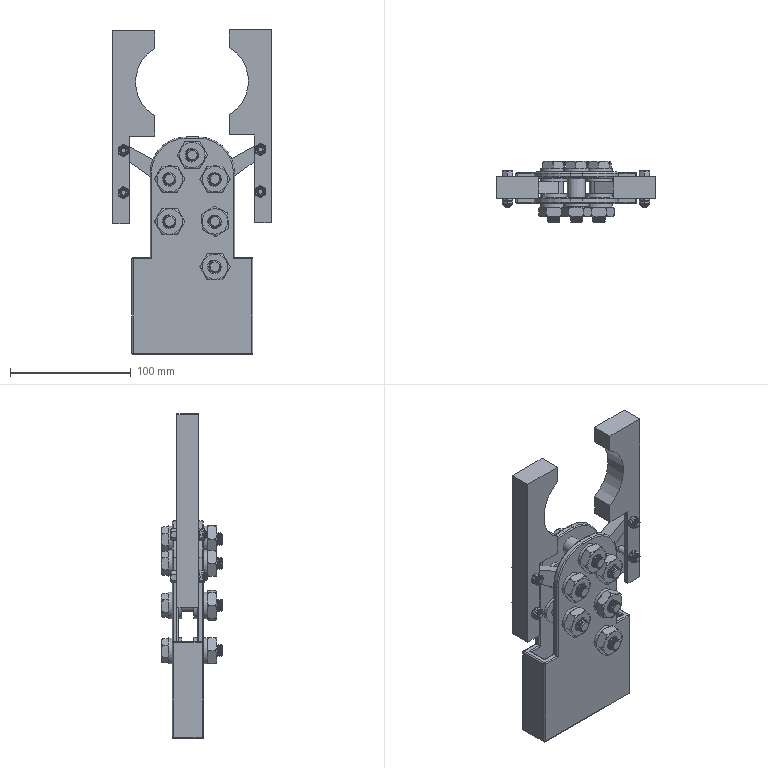Assembly | NX | mm | 50 component files | 60 solids | 643 faces | box 131.4 x 51 x 268.75 mm | volume 346007 mm3 | plane 296 | cylinder 247 | spline 40 | torus 38 | cone 14 | sphere 8 | commonest cylinder face diameters 10 x109 6 x49 2 x36 22 x24 8.5 x6 12 x6 5 x4 8 x4
Bill of materials:
unnamed part 1 | 2 |  | Flat tapered link or lever plate with rounded ends and two round through holes: a larger hole at the wide end and a smaller hole at the narrow end.
unnamed part 2 | 2 |  | Flat profiled plate: a wider upper portion with a large concave circular-arc cutout on one edge, then a step down to a narrower straight leg with two small round through holes along it.
unnamed part 3 | 4 |  | Hex-head bolt with a partially threaded shank: a plain cylindrical shank under the head and external threads toward the chamfered tip.
unnamed part 4 | 1 |  | Plain cylindrical tube, sleeve or spacer with a concentric through bore and flat ends.
unnamed part 5 | 4 |  | Hex nut with chamfered corners on both faces and a modeled internal thread. It is fairly tall relative to its width across flats.
unnamed part 6 | 1 |  | Clevis-like bracket: a rectangular hollow tube base whose two opposite long walls continue upward as parallel flat tabs with rounded tops. Each tab has a pattern of round through holes.
unnamed part 7 | 6 |  | Hex-head bolt with a partially threaded shank: a plain shank section under the head and external threads toward the tip.
unnamed part 8 | 24 |  | Plain flat washer: a thin annular disk with a concentric center hole.
unnamed part 9 | 6 |  | Hex nut of moderate or low height, chamfered on both faces, with a modeled internal thread.
Mates:
1. concentric | JJZ-003 2 edge | JJZ-010 22 edge
2. concentric | JJZ-010 23 edge | JJZ-003 1 edge
3. concentric | JJZ-004 2 edge | JJZ-003 2 edge
4. concentric | JJZ-004 1 edge | JJZ-003 1 edge
5. parallel | JJZ-004 1 edge | JJZ-004 2 edge
6. concentric | JJZ-006 6 edge | JJZ-010 16 edge
7. concentric | JJZ-010 15 edge | JJZ-005 6 edge
8. concentric | JJZ-005 5 edge | JJZ-010 13 edge
9. concentric | JJZ-010 12 edge | JJZ-005 4 edge
10. concentric | JJZ-010 14 edge | JJZ-005 3 edge
11. concentric | JJZ-006 5 edge | JJZ-010 9 edge
12. concentric | JJZ-010 11 edge | JJZ-006 4 edge
13. concentric | JJZ-010 10 edge | JJZ-006 3 edge
14. concentric | JJZ-001 1 edge | JJZ-010 16 edge
15. concentric | JJZ-010 8 edge | JJZ-001 1 edge
16. fix | JJZ-001 1 component
17. concentric | JJZ-001 1 edge | JJZ-010 7 edge
18. concentric | JJZ-001 1 edge | JJZ-010 6 edge
19. concentric | JJZ-001 1 edge | JJZ-010 5 edge
20. concentric | JJZ-005 2 edge | JJZ-010 6 edge
21. concentric | JJZ-010 5 edge | JJZ-005 1 edge
22. concentric | JJZ-006 2 edge | JJZ-010 7 edge
23. concentric | JJZ-006 1 edge | JJZ-010 8 edge
24. concentric | JJZ-001 1 edge | JJZ-010 4 edge
25. concentric | JJZ-001 1 edge | JJZ-010 3 edge
26. concentric | JJZ-007 1 edge | JJZ-001 1 edge
27. concentric | JJZ-004 2 edge | JJZ-008 4 edge
28. concentric | JJZ-004 1 edge | JJZ-008 3 edge
29. concentric | JJZ-004 1 edge | JJZ-008 2 edge
30. concentric | JJZ-008 1 edge | JJZ-004 2 edge
31. concentric | JJZ-009 4 edge | JJZ-004 2 edge
32. concentric | JJZ-009 3 edge | JJZ-004 1 edge
33. concentric | JJZ-009 2 edge | JJZ-004 1 edge
34. concentric | JJZ-009 1 edge | JJZ-004 2 edge
35. concentric | JJZ-010 2 edge | JJZ-001 1 edge
36. concentric | JJZ-010 1 edge | JJZ-001 1 edge